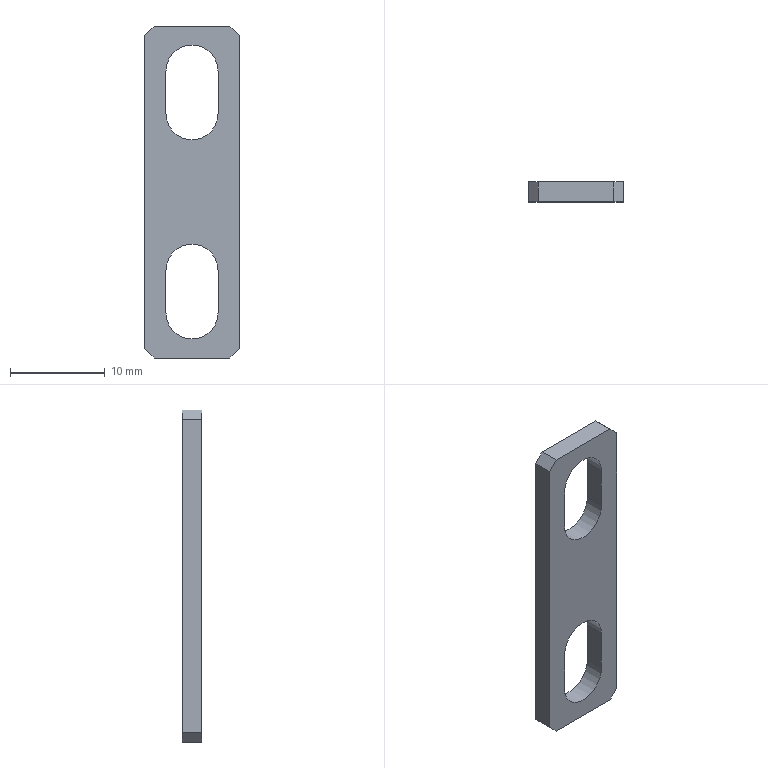Component | SolidWorks | 12-DividingMechanism-1111-1_20-1111-3 | 1 solid | 18 faces | box 10 x 2.1 x 35 mm | volume 527 mm3 | plane 14 | cylinder 4 | commonest cylinder face diameters 5.5 x4
STEP:
#1=COLOUR_RGB('',0.7922,0.8196,0.9333);
#2=FILL_AREA_STYLE_COLOUR('',#1);
#3=FILL_AREA_STYLE('',(#2));
#4=SURFACE_STYLE_FILL_AREA(#3);
#5=SURFACE_SIDE_STYLE('',(#4));
#6=SURFACE_STYLE_USAGE(.BOTH.,#5);
#7=PRESENTATION_STYLE_ASSIGNMENT((#6));
#8=CARTESIAN_POINT('',(2.044,22.592,60.967));
#9=VERTEX_POINT('',#8);
#10=CARTESIAN_POINT('',(2.359,22.592,60.967));
#11=VERTEX_POINT('',#10);
#12=CARTESIAN_POINT('',(2.399,22.592,60.967));
#13=DIRECTION('',(1.,-0.,0.));
#14=VECTOR('',#13,39.37);
#15=LINE('',#12,#14);
#16=EDGE_CURVE('',#9,#11,#15,.T.);
#17=ORIENTED_EDGE('',*,*,#16,.T.);
#18=CARTESIAN_POINT('',(2.359,22.674,60.967));
#19=VERTEX_POINT('',#18);
#20=CARTESIAN_POINT('',(2.359,22.674,60.967));
#21=DIRECTION('',(0.,1.,0.));
#22=VECTOR('',#21,39.37);
#23=LINE('',#20,#22);
#24=EDGE_CURVE('',#11,#19,#23,.T.);
#25=ORIENTED_EDGE('',*,*,#24,.T.);
#26=CARTESIAN_POINT('',(2.044,22.674,60.967));
#27=VERTEX_POINT('',#26);
#28=CARTESIAN_POINT('',(2.399,22.674,60.967));
#29=DIRECTION('',(1.,-0.,0.));
#30=VECTOR('',#29,39.37);
#31=LINE('',#28,#30);
#32=EDGE_CURVE('',#27,#19,#31,.T.);
#33=ORIENTED_EDGE('',*,*,#32,.F.);
#34=CARTESIAN_POINT('',(2.044,22.674,60.967));
#35=DIRECTION('',(-0.,-1.,-0.));
#36=VECTOR('',#35,39.37);
#37=LINE('',#34,#36);
#38=EDGE_CURVE('',#27,#9,#37,.T.);
#39=ORIENTED_EDGE('',*,*,#38,.T.);
#40=EDGE_LOOP('',(#17,#25,#33,#39));
#41=FACE_OUTER_BOUND('',#40,.T.);
#42=CARTESIAN_POINT('',(2.399,22.674,60.967));
#43=DIRECTION('',(0.,0.,-1.));
#44=DIRECTION('',(-1.,0.,-0.));
#45=AXIS2_PLACEMENT_3D('',#42,#43,#44);
#46=PLANE('',#45);
#47=ADVANCED_FACE('',(#41),#46,.F.);
#48=CARTESIAN_POINT('',(2.399,22.592,60.927));
#49=VERTEX_POINT('',#48);
#50=CARTESIAN_POINT('',(2.399,22.592,59.628));
#51=VERTEX_POINT('',#50);
#52=CARTESIAN_POINT('',(2.399,22.592,59.589));
#53=DIRECTION('',(0.,0.,-1.));
#54=VECTOR('',#53,39.37);
#55=LINE('',#52,#54);
#56=EDGE_CURVE('',#49,#51,#55,.T.);
#57=ORIENTED_EDGE('',*,*,#56,.T.);
#58=CARTESIAN_POINT('',(2.399,22.674,59.628));
#59=VERTEX_POINT('',#58);
#60=CARTESIAN_POINT('',(2.399,22.674,59.628));
#61=DIRECTION('',(0.,1.,0.));
#62=VECTOR('',#61,39.37);
#63=LINE('',#60,#62);
#64=EDGE_CURVE('',#51,#59,#63,.T.);
#65=ORIENTED_EDGE('',*,*,#64,.T.);
#66=CARTESIAN_POINT('',(2.399,22.674,60.927));
#67=VERTEX_POINT('',#66);
#68=CARTESIAN_POINT('',(2.399,22.674,59.589));
#69=DIRECTION('',(0.,0.,-1.));
#70=VECTOR('',#69,39.37);
#71=LINE('',#68,#70);
#72=EDGE_CURVE('',#67,#59,#71,.T.);
#73=ORIENTED_EDGE('',*,*,#72,.F.);
#74=CARTESIAN_POINT('',(2.399,22.674,60.927));
#75=DIRECTION('',(-0.,-1.,-0.));
#76=VECTOR('',#75,39.37);
#77=LINE('',#74,#76);
#78=EDGE_CURVE('',#67,#49,#77,.T.);
#79=ORIENTED_EDGE('',*,*,#78,.T.);
#80=EDGE_LOOP('',(#57,#65,#73,#79));
#81=FACE_OUTER_BOUND('',#80,.T.);
#82=CARTESIAN_POINT('',(2.399,22.674,59.589));
#83=DIRECTION('',(-1.,0.,-0.));
#84=DIRECTION('',(-0.,-0.,1.));
#85=AXIS2_PLACEMENT_3D('',#82,#83,#84);
#86=PLANE('',#85);
#87=ADVANCED_FACE('',(#81),#86,.F.);
#88=CARTESIAN_POINT('',(2.359,22.674,59.589));
#89=VERTEX_POINT('',#88);
#90=CARTESIAN_POINT('',(2.044,22.674,59.589));
#91=VERTEX_POINT('',#90);
#92=CARTESIAN_POINT('',(2.399,22.674,59.589));
#93=DIRECTION('',(-1.,0.,-0.));
#94=VECTOR('',#93,39.37);
#95=LINE('',#92,#94);
#96=EDGE_CURVE('',#89,#91,#95,.T.);
#97=ORIENTED_EDGE('',*,*,#96,.F.);
#98=CARTESIAN_POINT('',(2.359,22.592,59.589));
#99=VERTEX_POINT('',#98);
#100=CARTESIAN_POINT('',(2.359,22.674,59.589));
#101=DIRECTION('',(-0.,-1.,-0.));
#102=VECTOR('',#101,39.37);
#103=LINE('',#100,#102);
#104=EDGE_CURVE('',#89,#99,#103,.T.);
#105=ORIENTED_EDGE('',*,*,#104,.T.);
#106=CARTESIAN_POINT('',(2.044,22.592,59.589));
#107=VERTEX_POINT('',#106);
#108=CARTESIAN_POINT('',(2.399,22.592,59.589));
#109=DIRECTION('',(-1.,0.,-0.));
#110=VECTOR('',#109,39.37);
#111=LINE('',#108,#110);
#112=EDGE_CURVE('',#99,#107,#111,.T.);
#113=ORIENTED_EDGE('',*,*,#112,.T.);
#114=CARTESIAN_POINT('',(2.044,22.674,59.589));
#115=DIRECTION('',(0.,1.,0.));
#116=VECTOR('',#115,39.37);
#117=LINE('',#114,#116);
#118=EDGE_CURVE('',#107,#91,#117,.T.);
#119=ORIENTED_EDGE('',*,*,#118,.T.);
#120=EDGE_LOOP('',(#97,#105,#113,#119));
#121=FACE_OUTER_BOUND('',#120,.T.);
#122=CARTESIAN_POINT('',(2.399,22.674,59.589));
#123=DIRECTION('',(-0.,-0.,1.));
#124=DIRECTION('',(1.,-0.,0.));
#125=AXIS2_PLACEMENT_3D('',#122,#123,#124);
#126=PLANE('',#125);
#127=ADVANCED_FACE('',(#121),#126,.F.);
#128=CARTESIAN_POINT('',(2.005,22.674,60.927));
#129=VERTEX_POINT('',#128);
#130=CARTESIAN_POINT('',(2.005,22.674,59.628));
#131=VERTEX_POINT('',#130);
#132=CARTESIAN_POINT('',(2.005,22.674,59.097));
#133=DIRECTION('',(0.,0.,-1.));
#134=VECTOR('',#133,39.37);
#135=LINE('',#132,#134);
#136=EDGE_CURVE('',#129,#131,#135,.T.);
#137=ORIENTED_EDGE('',*,*,#136,.F.);
#138=CARTESIAN_POINT('',(0.7452,22.674,59.668));
#139=DIRECTION('',(0.7071,-0.,0.7071));
#140=VECTOR('',#139,39.37);
#141=LINE('',#138,#140);
#142=EDGE_CURVE('',#129,#27,#141,.T.);
#143=ORIENTED_EDGE('',*,*,#142,.T.);
#144=ORIENTED_EDGE('',*,*,#32,.T.);
#145=CARTESIAN_POINT('',(1.592,22.674,61.734));
#146=DIRECTION('',(0.7071,-0.,-0.7071));
#147=VECTOR('',#146,39.37);
#148=LINE('',#145,#147);
#149=EDGE_CURVE('',#19,#67,#148,.T.);
#150=ORIENTED_EDGE('',*,*,#149,.T.);
#151=ORIENTED_EDGE('',*,*,#72,.T.);
#152=CARTESIAN_POINT('',(1.592,22.674,58.821));
#153=DIRECTION('',(-0.7071,0.,-0.7071));
#154=VECTOR('',#153,39.37);
#155=LINE('',#152,#154);
#156=EDGE_CURVE('',#59,#89,#155,.T.);
#157=ORIENTED_EDGE('',*,*,#156,.T.);
#158=ORIENTED_EDGE('',*,*,#96,.T.);
#159=CARTESIAN_POINT('',(0.7452,22.674,60.888));
#160=DIRECTION('',(-0.7071,0.,0.7071));
#161=VECTOR('',#160,39.37);
#162=LINE('',#159,#161);
#163=EDGE_CURVE('',#91,#131,#162,.T.);
#164=ORIENTED_EDGE('',*,*,#163,.T.);
#165=EDGE_LOOP('',(#137,#143,#144,#150,#151,#157,#158,#164));
#166=FACE_OUTER_BOUND('',#165,.T.);
#167=CARTESIAN_POINT('',(2.31,22.674,59.953));
#168=VERTEX_POINT('',#167);
#169=CARTESIAN_POINT('',(2.31,22.674,59.776));
#170=VERTEX_POINT('',#169);
#171=CARTESIAN_POINT('',(2.31,22.674,59.953));
#172=DIRECTION('',(0.,0.,-1.));
#173=VECTOR('',#172,39.37);
#174=LINE('',#171,#173);
#175=EDGE_CURVE('',#168,#170,#174,.T.);
#176=ORIENTED_EDGE('',*,*,#175,.F.);
#177=CARTESIAN_POINT('',(2.094,22.674,59.953));
#178=VERTEX_POINT('',#177);
#179=CARTESIAN_POINT('',(2.202,22.674,59.953));
#180=DIRECTION('',(0.,1.,0.));
#181=DIRECTION('',(1.,0.,0.));
#182=AXIS2_PLACEMENT_3D('',#179,#180,#181);
#183=CIRCLE('',#182,0.1083);
#184=EDGE_CURVE('',#178,#168,#183,.T.);
#185=ORIENTED_EDGE('',*,*,#184,.F.);
#186=CARTESIAN_POINT('',(2.094,22.674,59.776));
#187=VERTEX_POINT('',#186);
#188=CARTESIAN_POINT('',(2.094,22.674,59.953));
#189=DIRECTION('',(0.,0.,-1.));
#190=VECTOR('',#189,39.37);
#191=LINE('',#188,#190);
#192=EDGE_CURVE('',#178,#187,#191,.T.);
#193=ORIENTED_EDGE('',*,*,#192,.T.);
#194=CARTESIAN_POINT('',(2.202,22.674,59.776));
#195=DIRECTION('',(0.,1.,0.));
#196=DIRECTION('',(1.,0.,0.));
#197=AXIS2_PLACEMENT_3D('',#194,#195,#196);
#198=CIRCLE('',#197,0.1083);
#199=EDGE_CURVE('',#170,#187,#198,.T.);
#200=ORIENTED_EDGE('',*,*,#199,.F.);
#201=EDGE_LOOP('',(#176,#185,#193,#200));
#202=FACE_BOUND('',#201,.T.);
#203=CARTESIAN_POINT('',(2.31,22.674,60.78));
#204=VERTEX_POINT('',#203);
#205=CARTESIAN_POINT('',(2.31,22.674,60.603));
#206=VERTEX_POINT('',#205);
#207=CARTESIAN_POINT('',(2.31,22.674,60.78));
#208=DIRECTION('',(0.,0.,-1.));
#209=VECTOR('',#208,39.37);
#210=LINE('',#207,#209);
#211=EDGE_CURVE('',#204,#206,#210,.T.);
#212=ORIENTED_EDGE('',*,*,#211,.F.);
#213=CARTESIAN_POINT('',(2.094,22.674,60.78));
#214=VERTEX_POINT('',#213);
#215=CARTESIAN_POINT('',(2.202,22.674,60.78));
#216=DIRECTION('',(0.,1.,0.));
#217=DIRECTION('',(1.,0.,0.));
#218=AXIS2_PLACEMENT_3D('',#215,#216,#217);
#219=CIRCLE('',#218,0.1083);
#220=EDGE_CURVE('',#214,#204,#219,.T.);
#221=ORIENTED_EDGE('',*,*,#220,.F.);
#222=CARTESIAN_POINT('',(2.094,22.674,60.603));
#223=VERTEX_POINT('',#222);
#224=CARTESIAN_POINT('',(2.094,22.674,60.78));
#225=DIRECTION('',(0.,0.,-1.));
#226=VECTOR('',#225,39.37);
#227=LINE('',#224,#226);
#228=EDGE_CURVE('',#214,#223,#227,.T.);
#229=ORIENTED_EDGE('',*,*,#228,.T.);
#230=CARTESIAN_POINT('',(2.202,22.674,60.603));
#231=DIRECTION('',(0.,1.,0.));
#232=DIRECTION('',(1.,0.,0.));
#233=AXIS2_PLACEMENT_3D('',#230,#231,#232);
#234=CIRCLE('',#233,0.1083);
#235=EDGE_CURVE('',#206,#223,#234,.T.);
#236=ORIENTED_EDGE('',*,*,#235,.F.);
#237=EDGE_LOOP('',(#212,#221,#229,#236));
#238=FACE_BOUND('',#237,.T.);
#239=CARTESIAN_POINT('',(0.135,22.674,60.278));
#240=DIRECTION('',(0.,1.,0.));
#241=DIRECTION('',(1.,-0.,0.));
#242=AXIS2_PLACEMENT_3D('',#239,#240,#241);
#243=PLANE('',#242);
#244=ADVANCED_FACE('',(#166,#202,#238),#243,.T.);
#245=CARTESIAN_POINT('',(2.31,22.592,59.953));
#246=VERTEX_POINT('',#245);
#247=CARTESIAN_POINT('',(2.31,22.592,59.776));
#248=VERTEX_POINT('',#247);
#249=CARTESIAN_POINT('',(2.31,22.592,59.953));
#250=DIRECTION('',(0.,0.,-1.));
#251=VECTOR('',#250,39.37);
#252=LINE('',#249,#251);
#253=EDGE_CURVE('',#246,#248,#252,.T.);
#254=ORIENTED_EDGE('',*,*,#253,.T.);
#255=CARTESIAN_POINT('',(2.094,22.592,59.776));
#256=VERTEX_POINT('',#255);
#257=CARTESIAN_POINT('',(2.202,22.592,59.776));
#258=DIRECTION('',(0.,1.,0.));
#259=DIRECTION('',(1.,0.,0.));
#260=AXIS2_PLACEMENT_3D('',#257,#258,#259);
#261=CIRCLE('',#260,0.1083);
#262=EDGE_CURVE('',#248,#256,#261,.T.);
#263=ORIENTED_EDGE('',*,*,#262,.T.);
#264=CARTESIAN_POINT('',(2.094,22.592,59.953));
#265=VERTEX_POINT('',#264);
#266=CARTESIAN_POINT('',(2.094,22.592,59.953));
#267=DIRECTION('',(0.,0.,-1.));
#268=VECTOR('',#267,39.37);
#269=LINE('',#266,#268);
#270=EDGE_CURVE('',#265,#256,#269,.T.);
#271=ORIENTED_EDGE('',*,*,#270,.F.);
#272=CARTESIAN_POINT('',(2.202,22.592,59.953));
#273=DIRECTION('',(0.,1.,0.));
#274=DIRECTION('',(1.,0.,0.));
#275=AXIS2_PLACEMENT_3D('',#272,#273,#274);
#276=CIRCLE('',#275,0.1083);
#277=EDGE_CURVE('',#265,#246,#276,.T.);
#278=ORIENTED_EDGE('',*,*,#277,.T.);
#279=EDGE_LOOP('',(#254,#263,#271,#278));
#280=FACE_BOUND('',#279,.T.);
#281=CARTESIAN_POINT('',(2.094,22.592,60.78));
#282=VERTEX_POINT('',#281);
#283=CARTESIAN_POINT('',(2.094,22.592,60.603));
#284=VERTEX_POINT('',#283);
#285=CARTESIAN_POINT('',(2.094,22.592,60.78));
#286=DIRECTION('',(0.,0.,-1.));
#287=VECTOR('',#286,39.37);
#288=LINE('',#285,#287);
#289=EDGE_CURVE('',#282,#284,#288,.T.);
#290=ORIENTED_EDGE('',*,*,#289,.F.);
#291=CARTESIAN_POINT('',(2.31,22.592,60.78));
#292=VERTEX_POINT('',#291);
#293=CARTESIAN_POINT('',(2.202,22.592,60.78));
#294=DIRECTION('',(0.,1.,0.));
#295=DIRECTION('',(1.,0.,0.));
#296=AXIS2_PLACEMENT_3D('',#293,#294,#295);
#297=CIRCLE('',#296,0.1083);
#298=EDGE_CURVE('',#282,#292,#297,.T.);
#299=ORIENTED_EDGE('',*,*,#298,.T.);
#300=CARTESIAN_POINT('',(2.31,22.592,60.603));
#301=VERTEX_POINT('',#300);
#302=CARTESIAN_POINT('',(2.31,22.592,60.78));
#303=DIRECTION('',(0.,0.,-1.));
#304=VECTOR('',#303,39.37);
#305=LINE('',#302,#304);
#306=EDGE_CURVE('',#292,#301,#305,.T.);
#307=ORIENTED_EDGE('',*,*,#306,.T.);
#308=CARTESIAN_POINT('',(2.202,22.592,60.603));
#309=DIRECTION('',(0.,1.,0.));
#310=DIRECTION('',(1.,0.,0.));
#311=AXIS2_PLACEMENT_3D('',#308,#309,#310);
#312=CIRCLE('',#311,0.1083);
#313=EDGE_CURVE('',#301,#284,#312,.T.);
#314=ORIENTED_EDGE('',*,*,#313,.T.);
#315=EDGE_LOOP('',(#290,#299,#307,#314));
#316=FACE_BOUND('',#315,.T.);
#317=CARTESIAN_POINT('',(2.005,22.592,60.927));
#318=VERTEX_POINT('',#317);
#319=CARTESIAN_POINT('',(2.044,22.592,60.967));
#320=DIRECTION('',(-0.7071,0.,-0.7071));
#321=VECTOR('',#320,39.37);
#322=LINE('',#319,#321);
#323=EDGE_CURVE('',#9,#318,#322,.T.);
#324=ORIENTED_EDGE('',*,*,#323,.T.);
#325=CARTESIAN_POINT('',(2.005,22.592,59.628));
#326=VERTEX_POINT('',#325);
#327=CARTESIAN_POINT('',(2.005,22.592,59.097));
#328=DIRECTION('',(0.,0.,-1.));
#329=VECTOR('',#328,39.37);
#330=LINE('',#327,#329);
#331=EDGE_CURVE('',#318,#326,#330,.T.);
#332=ORIENTED_EDGE('',*,*,#331,.T.);
#333=CARTESIAN_POINT('',(2.044,22.592,59.589));
#334=DIRECTION('',(0.7071,-0.,-0.7071));
#335=VECTOR('',#334,39.37);
#336=LINE('',#333,#335);
#337=EDGE_CURVE('',#326,#107,#336,.T.);
#338=ORIENTED_EDGE('',*,*,#337,.T.);
#339=ORIENTED_EDGE('',*,*,#112,.F.);
#340=CARTESIAN_POINT('',(2.359,22.592,59.589));
#341=DIRECTION('',(0.7071,-0.,0.7071));
#342=VECTOR('',#341,39.37);
#343=LINE('',#340,#342);
#344=EDGE_CURVE('',#99,#51,#343,.T.);
#345=ORIENTED_EDGE('',*,*,#344,.T.);
#346=ORIENTED_EDGE('',*,*,#56,.F.);
#347=CARTESIAN_POINT('',(2.399,22.592,60.927));
#348=DIRECTION('',(-0.7071,0.,0.7071));
#349=VECTOR('',#348,39.37);
#350=LINE('',#347,#349);
#351=EDGE_CURVE('',#49,#11,#350,.T.);
#352=ORIENTED_EDGE('',*,*,#351,.T.);
#353=ORIENTED_EDGE('',*,*,#16,.F.);
#354=EDGE_LOOP('',(#324,#332,#338,#339,#345,#346,#352,#353));
#355=FACE_OUTER_BOUND('',#354,.T.);
#356=CARTESIAN_POINT('',(0.135,22.592,60.278));
#357=DIRECTION('',(0.,1.,0.));
#358=DIRECTION('',(1.,-0.,0.));
#359=AXIS2_PLACEMENT_3D('',#356,#357,#358);
#360=PLANE('',#359);
#361=ADVANCED_FACE('',(#280,#316,#355),#360,.F.);
#362=ORIENTED_EDGE('',*,*,#136,.T.);
#363=CARTESIAN_POINT('',(2.005,22.592,59.628));
#364=DIRECTION('',(-0.,-1.,-0.));
#365=VECTOR('',#364,39.37);
#366=LINE('',#363,#365);
#367=EDGE_CURVE('',#131,#326,#366,.T.);
#368=ORIENTED_EDGE('',*,*,#367,.T.);
#369=ORIENTED_EDGE('',*,*,#331,.F.);
#370=CARTESIAN_POINT('',(2.005,22.592,60.927));
#371=DIRECTION('',(0.,1.,0.));
#372=VECTOR('',#371,39.37);
#373=LINE('',#370,#372);
#374=EDGE_CURVE('',#318,#129,#373,.T.);
#375=ORIENTED_EDGE('',*,*,#374,.T.);
#376=EDGE_LOOP('',(#362,#368,#369,#375));
#377=FACE_OUTER_BOUND('',#376,.T.);
#378=CARTESIAN_POINT('',(2.005,22.592,59.097));
#379=DIRECTION('',(1.,-0.,0.));
#380=DIRECTION('',(0.,0.,-1.));
#381=AXIS2_PLACEMENT_3D('',#378,#379,#380);
#382=PLANE('',#381);
#383=ADVANCED_FACE('',(#377),#382,.F.);
#384=ORIENTED_EDGE('',*,*,#313,.F.);
#385=CARTESIAN_POINT('',(2.31,22.674,60.603));
#386=DIRECTION('',(-0.,-1.,-0.));
#387=VECTOR('',#386,39.37);
#388=LINE('',#385,#387);
#389=EDGE_CURVE('',#206,#301,#388,.T.);
#390=ORIENTED_EDGE('',*,*,#389,.F.);
#391=ORIENTED_EDGE('',*,*,#235,.T.);
#392=CARTESIAN_POINT('',(2.094,22.674,60.603));
#393=DIRECTION('',(0.,1.,0.));
#394=VECTOR('',#393,39.37);
#395=LINE('',#392,#394);
#396=EDGE_CURVE('',#284,#223,#395,.T.);
#397=ORIENTED_EDGE('',*,*,#396,.F.);
#398=EDGE_LOOP('',(#384,#390,#391,#397));
#399=FACE_OUTER_BOUND('',#398,.T.);
#400=CARTESIAN_POINT('',(2.202,22.674,60.603));
#401=DIRECTION('',(0.,1.,0.));
#402=DIRECTION('',(1.,0.,0.));
#403=AXIS2_PLACEMENT_3D('',#400,#401,#402);
#404=CYLINDRICAL_SURFACE('',#403,0.1083);
#405=ADVANCED_FACE('',(#399),#404,.F.);
#406=ORIENTED_EDGE('',*,*,#220,.T.);
#407=CARTESIAN_POINT('',(2.31,22.674,60.78));
#408=DIRECTION('',(0.,1.,0.));
#409=VECTOR('',#408,39.37);
#410=LINE('',#407,#409);
#411=EDGE_CURVE('',#292,#204,#410,.T.);
#412=ORIENTED_EDGE('',*,*,#411,.F.);
#413=ORIENTED_EDGE('',*,*,#298,.F.);
#414=CARTESIAN_POINT('',(2.094,22.674,60.78));
#415=DIRECTION('',(-0.,-1.,-0.));
#416=VECTOR('',#415,39.37);
#417=LINE('',#414,#416);
#418=EDGE_CURVE('',#214,#282,#417,.T.);
#419=ORIENTED_EDGE('',*,*,#418,.F.);
#420=EDGE_LOOP('',(#406,#412,#413,#419));
#421=FACE_OUTER_BOUND('',#420,.T.);
#422=CARTESIAN_POINT('',(2.202,22.674,60.78));
#423=DIRECTION('',(0.,1.,0.));
#424=DIRECTION('',(1.,0.,0.));
#425=AXIS2_PLACEMENT_3D('',#422,#423,#424);
#426=CYLINDRICAL_SURFACE('',#425,0.1083);
#427=ADVANCED_FACE('',(#421),#426,.F.);
#428=ORIENTED_EDGE('',*,*,#396,.T.);
#429=ORIENTED_EDGE('',*,*,#228,.F.);
#430=ORIENTED_EDGE('',*,*,#418,.T.);
#431=ORIENTED_EDGE('',*,*,#289,.T.);
#432=EDGE_LOOP('',(#428,#429,#430,#431));
#433=FACE_OUTER_BOUND('',#432,.T.);
#434=CARTESIAN_POINT('',(2.094,22.674,60.78));
#435=DIRECTION('',(-1.,0.,-0.));
#436=DIRECTION('',(-0.,-0.,1.));
#437=AXIS2_PLACEMENT_3D('',#434,#435,#436);
#438=PLANE('',#437);
#439=ADVANCED_FACE('',(#433),#438,.F.);
#440=ORIENTED_EDGE('',*,*,#389,.T.);
#441=ORIENTED_EDGE('',*,*,#306,.F.);
#442=ORIENTED_EDGE('',*,*,#411,.T.);
#443=ORIENTED_EDGE('',*,*,#211,.T.);
#444=EDGE_LOOP('',(#440,#441,#442,#443));
#445=FACE_OUTER_BOUND('',#444,.T.);
#446=CARTESIAN_POINT('',(2.31,22.674,60.78));
#447=DIRECTION('',(1.,-0.,0.));
#448=DIRECTION('',(0.,0.,-1.));
#449=AXIS2_PLACEMENT_3D('',#446,#447,#448);
#450=PLANE('',#449);
#451=ADVANCED_FACE('',(#445),#450,.F.);
#452=ORIENTED_EDGE('',*,*,#262,.F.);
#453=CARTESIAN_POINT('',(2.31,22.674,59.776));
#454=DIRECTION('',(-0.,-1.,-0.));
#455=VECTOR('',#454,39.37);
#456=LINE('',#453,#455);
#457=EDGE_CURVE('',#170,#248,#456,.T.);
#458=ORIENTED_EDGE('',*,*,#457,.F.);
#459=ORIENTED_EDGE('',*,*,#199,.T.);
#460=CARTESIAN_POINT('',(2.094,22.674,59.776));
#461=DIRECTION('',(0.,1.,0.));
#462=VECTOR('',#461,39.37);
#463=LINE('',#460,#462);
#464=EDGE_CURVE('',#256,#187,#463,.T.);
#465=ORIENTED_EDGE('',*,*,#464,.F.);
#466=EDGE_LOOP('',(#452,#458,#459,#465));
#467=FACE_OUTER_BOUND('',#466,.T.);
#468=CARTESIAN_POINT('',(2.202,22.674,59.776));
#469=DIRECTION('',(0.,1.,0.));
#470=DIRECTION('',(1.,0.,0.));
#471=AXIS2_PLACEMENT_3D('',#468,#469,#470);
#472=CYLINDRICAL_SURFACE('',#471,0.1083);
#473=ADVANCED_FACE('',(#467),#472,.F.);
#474=ORIENTED_EDGE('',*,*,#184,.T.);
#475=CARTESIAN_POINT('',(2.31,22.674,59.953));
#476=DIRECTION('',(0.,1.,0.));
#477=VECTOR('',#476,39.37);
#478=LINE('',#475,#477);
#479=EDGE_CURVE('',#246,#168,#478,.T.);
#480=ORIENTED_EDGE('',*,*,#479,.F.);
#481=ORIENTED_EDGE('',*,*,#277,.F.);
#482=CARTESIAN_POINT('',(2.094,22.674,59.953));
#483=DIRECTION('',(-0.,-1.,-0.));
#484=VECTOR('',#483,39.37);
#485=LINE('',#482,#484);
#486=EDGE_CURVE('',#178,#265,#485,.T.);
#487=ORIENTED_EDGE('',*,*,#486,.F.);
#488=EDGE_LOOP('',(#474,#480,#481,#487));
#489=FACE_OUTER_BOUND('',#488,.T.);
#490=CARTESIAN_POINT('',(2.202,22.674,59.953));
#491=DIRECTION('',(0.,1.,0.));
#492=DIRECTION('',(1.,0.,0.));
#493=AXIS2_PLACEMENT_3D('',#490,#491,#492);
#494=CYLINDRICAL_SURFACE('',#493,0.1083);
#495=ADVANCED_FACE('',(#489),#494,.F.);
#496=ORIENTED_EDGE('',*,*,#464,.T.);
#497=ORIENTED_EDGE('',*,*,#192,.F.);
#498=ORIENTED_EDGE('',*,*,#486,.T.);
#499=ORIENTED_EDGE('',*,*,#270,.T.);
#500=EDGE_LOOP('',(#496,#497,#498,#499));
#501=FACE_OUTER_BOUND('',#500,.T.);
#502=CARTESIAN_POINT('',(2.094,22.674,59.953));
#503=DIRECTION('',(-1.,0.,-0.));
#504=DIRECTION('',(-0.,-0.,1.));
#505=AXIS2_PLACEMENT_3D('',#502,#503,#504);
#506=PLANE('',#505);
#507=ADVANCED_FACE('',(#501),#506,.F.);
#508=ORIENTED_EDGE('',*,*,#457,.T.);
#509=ORIENTED_EDGE('',*,*,#253,.F.);
#510=ORIENTED_EDGE('',*,*,#479,.T.);
#511=ORIENTED_EDGE('',*,*,#175,.T.);
#512=EDGE_LOOP('',(#508,#509,#510,#511));
#513=FACE_OUTER_BOUND('',#512,.T.);
#514=CARTESIAN_POINT('',(2.31,22.674,59.953));
#515=DIRECTION('',(1.,-0.,0.));
#516=DIRECTION('',(0.,0.,-1.));
#517=AXIS2_PLACEMENT_3D('',#514,#515,#516);
#518=PLANE('',#517);
#519=ADVANCED_FACE('',(#513),#518,.F.);
#520=ORIENTED_EDGE('',*,*,#156,.F.);
#521=ORIENTED_EDGE('',*,*,#64,.F.);
#522=ORIENTED_EDGE('',*,*,#344,.F.);
#523=ORIENTED_EDGE('',*,*,#104,.F.);
#524=EDGE_LOOP('',(#520,#521,#522,#523));
#525=FACE_OUTER_BOUND('',#524,.T.);
#526=CARTESIAN_POINT('',(2.359,22.674,59.589));
#527=DIRECTION('',(-0.7071,0.,0.7071));
#528=DIRECTION('',(-0.,-1.,-0.));
#529=AXIS2_PLACEMENT_3D('',#526,#527,#528);
#530=PLANE('',#529);
#531=ADVANCED_FACE('',(#525),#530,.F.);
#532=ORIENTED_EDGE('',*,*,#337,.F.);
#533=ORIENTED_EDGE('',*,*,#367,.F.);
#534=ORIENTED_EDGE('',*,*,#163,.F.);
#535=ORIENTED_EDGE('',*,*,#118,.F.);
#536=EDGE_LOOP('',(#532,#533,#534,#535));
#537=FACE_OUTER_BOUND('',#536,.T.);
#538=CARTESIAN_POINT('',(2.044,22.674,59.589));
#539=DIRECTION('',(0.7071,-0.,0.7071));
#540=DIRECTION('',(0.,1.,0.));
#541=AXIS2_PLACEMENT_3D('',#538,#539,#540);
#542=PLANE('',#541);
#543=ADVANCED_FACE('',(#537),#542,.F.);
#544=ORIENTED_EDGE('',*,*,#149,.F.);
#545=ORIENTED_EDGE('',*,*,#24,.F.);
#546=ORIENTED_EDGE('',*,*,#351,.F.);
#547=ORIENTED_EDGE('',*,*,#78,.F.);
#548=EDGE_LOOP('',(#544,#545,#546,#547));
#549=FACE_OUTER_BOUND('',#548,.T.);
#550=CARTESIAN_POINT('',(2.399,22.674,60.927));
#551=DIRECTION('',(-0.7071,0.,-0.7071));
#552=DIRECTION('',(-0.,-1.,-0.));
#553=AXIS2_PLACEMENT_3D('',#550,#551,#552);
#554=PLANE('',#553);
#555=ADVANCED_FACE('',(#549),#554,.F.);
#556=ORIENTED_EDGE('',*,*,#142,.F.);
#557=ORIENTED_EDGE('',*,*,#374,.F.);
#558=ORIENTED_EDGE('',*,*,#323,.F.);
#559=ORIENTED_EDGE('',*,*,#38,.F.);
#560=EDGE_LOOP('',(#556,#557,#558,#559));
#561=FACE_OUTER_BOUND('',#560,.T.);
#562=CARTESIAN_POINT('',(2.044,22.674,60.967));
#563=DIRECTION('',(0.7071,-0.,-0.7071));
#564=DIRECTION('',(-0.,-1.,-0.));
#565=AXIS2_PLACEMENT_3D('',#562,#563,#564);
#566=PLANE('',#565);
#567=ADVANCED_FACE('',(#561),#566,.F.);
#568=CLOSED_SHELL('',(#47,#87,#127,#244,#361,#383,#405,#427,#439,#451,#473,#495,#507,#519,#531,#543,#555,#567));
#569=MANIFOLD_SOLID_BREP('',#568);
#570=STYLED_ITEM('',(#7),#569);
#571=PRESENTATION_LAYER_ASSIGNMENT('','',(#570));
#572=(LENGTH_UNIT()NAMED_UNIT(*)SI_UNIT($,.METRE.));
#573=LENGTH_MEASURE_WITH_UNIT(LENGTH_MEASURE(0.0254),#572);
#574=DIMENSIONAL_EXPONENTS(1.,0.,0.,0.,0.,0.,0.);
#575=(CONVERSION_BASED_UNIT('',#573)LENGTH_UNIT()NAMED_UNIT(#574));
#576=UNCERTAINTY_MEASURE_WITH_UNIT(LENGTH_MEASURE(0.00001),#575,'','');
#577=(NAMED_UNIT(*)PLANE_ANGLE_UNIT()SI_UNIT($,.RADIAN.));
#578=(NAMED_UNIT(*)SI_UNIT($,.STERADIAN.)SOLID_ANGLE_UNIT());
#579=(GEOMETRIC_REPRESENTATION_CONTEXT(3)GLOBAL_UNCERTAINTY_ASSIGNED_CONTEXT((#576))GLOBAL_UNIT_ASSIGNED_CONTEXT((#575,#577,#578))REPRESENTATION_CONTEXT('',''));
#580=MECHANICAL_DESIGN_GEOMETRIC_PRESENTATION_REPRESENTATION('',(#570),#579);
#581=CARTESIAN_POINT('',(0.,0.,0.));
#582=DIRECTION('',(0.,0.,1.));
#583=DIRECTION('',(1.,0.,0.));
#584=AXIS2_PLACEMENT_3D('',#581,#582,#583);
#585=(LENGTH_UNIT()NAMED_UNIT(*)SI_UNIT($,.METRE.));
#586=LENGTH_MEASURE_WITH_UNIT(LENGTH_MEASURE(0.0254),#585);
#587=DIMENSIONAL_EXPONENTS(1.,0.,0.,0.,0.,0.,0.);
#588=(CONVERSION_BASED_UNIT('',#586)LENGTH_UNIT()NAMED_UNIT(#587));
#589=UNCERTAINTY_MEASURE_WITH_UNIT(LENGTH_MEASURE(0.00001),#588,'','');
#590=(NAMED_UNIT(*)PLANE_ANGLE_UNIT()SI_UNIT($,.RADIAN.));
#591=(NAMED_UNIT(*)SI_UNIT($,.STERADIAN.)SOLID_ANGLE_UNIT());
#592=(GEOMETRIC_REPRESENTATION_CONTEXT(3)GLOBAL_UNCERTAINTY_ASSIGNED_CONTEXT((#589))GLOBAL_UNIT_ASSIGNED_CONTEXT((#588,#590,#591))REPRESENTATION_CONTEXT('',''));
#593=ADVANCED_BREP_SHAPE_REPRESENTATION('',(#569,#584),#592);